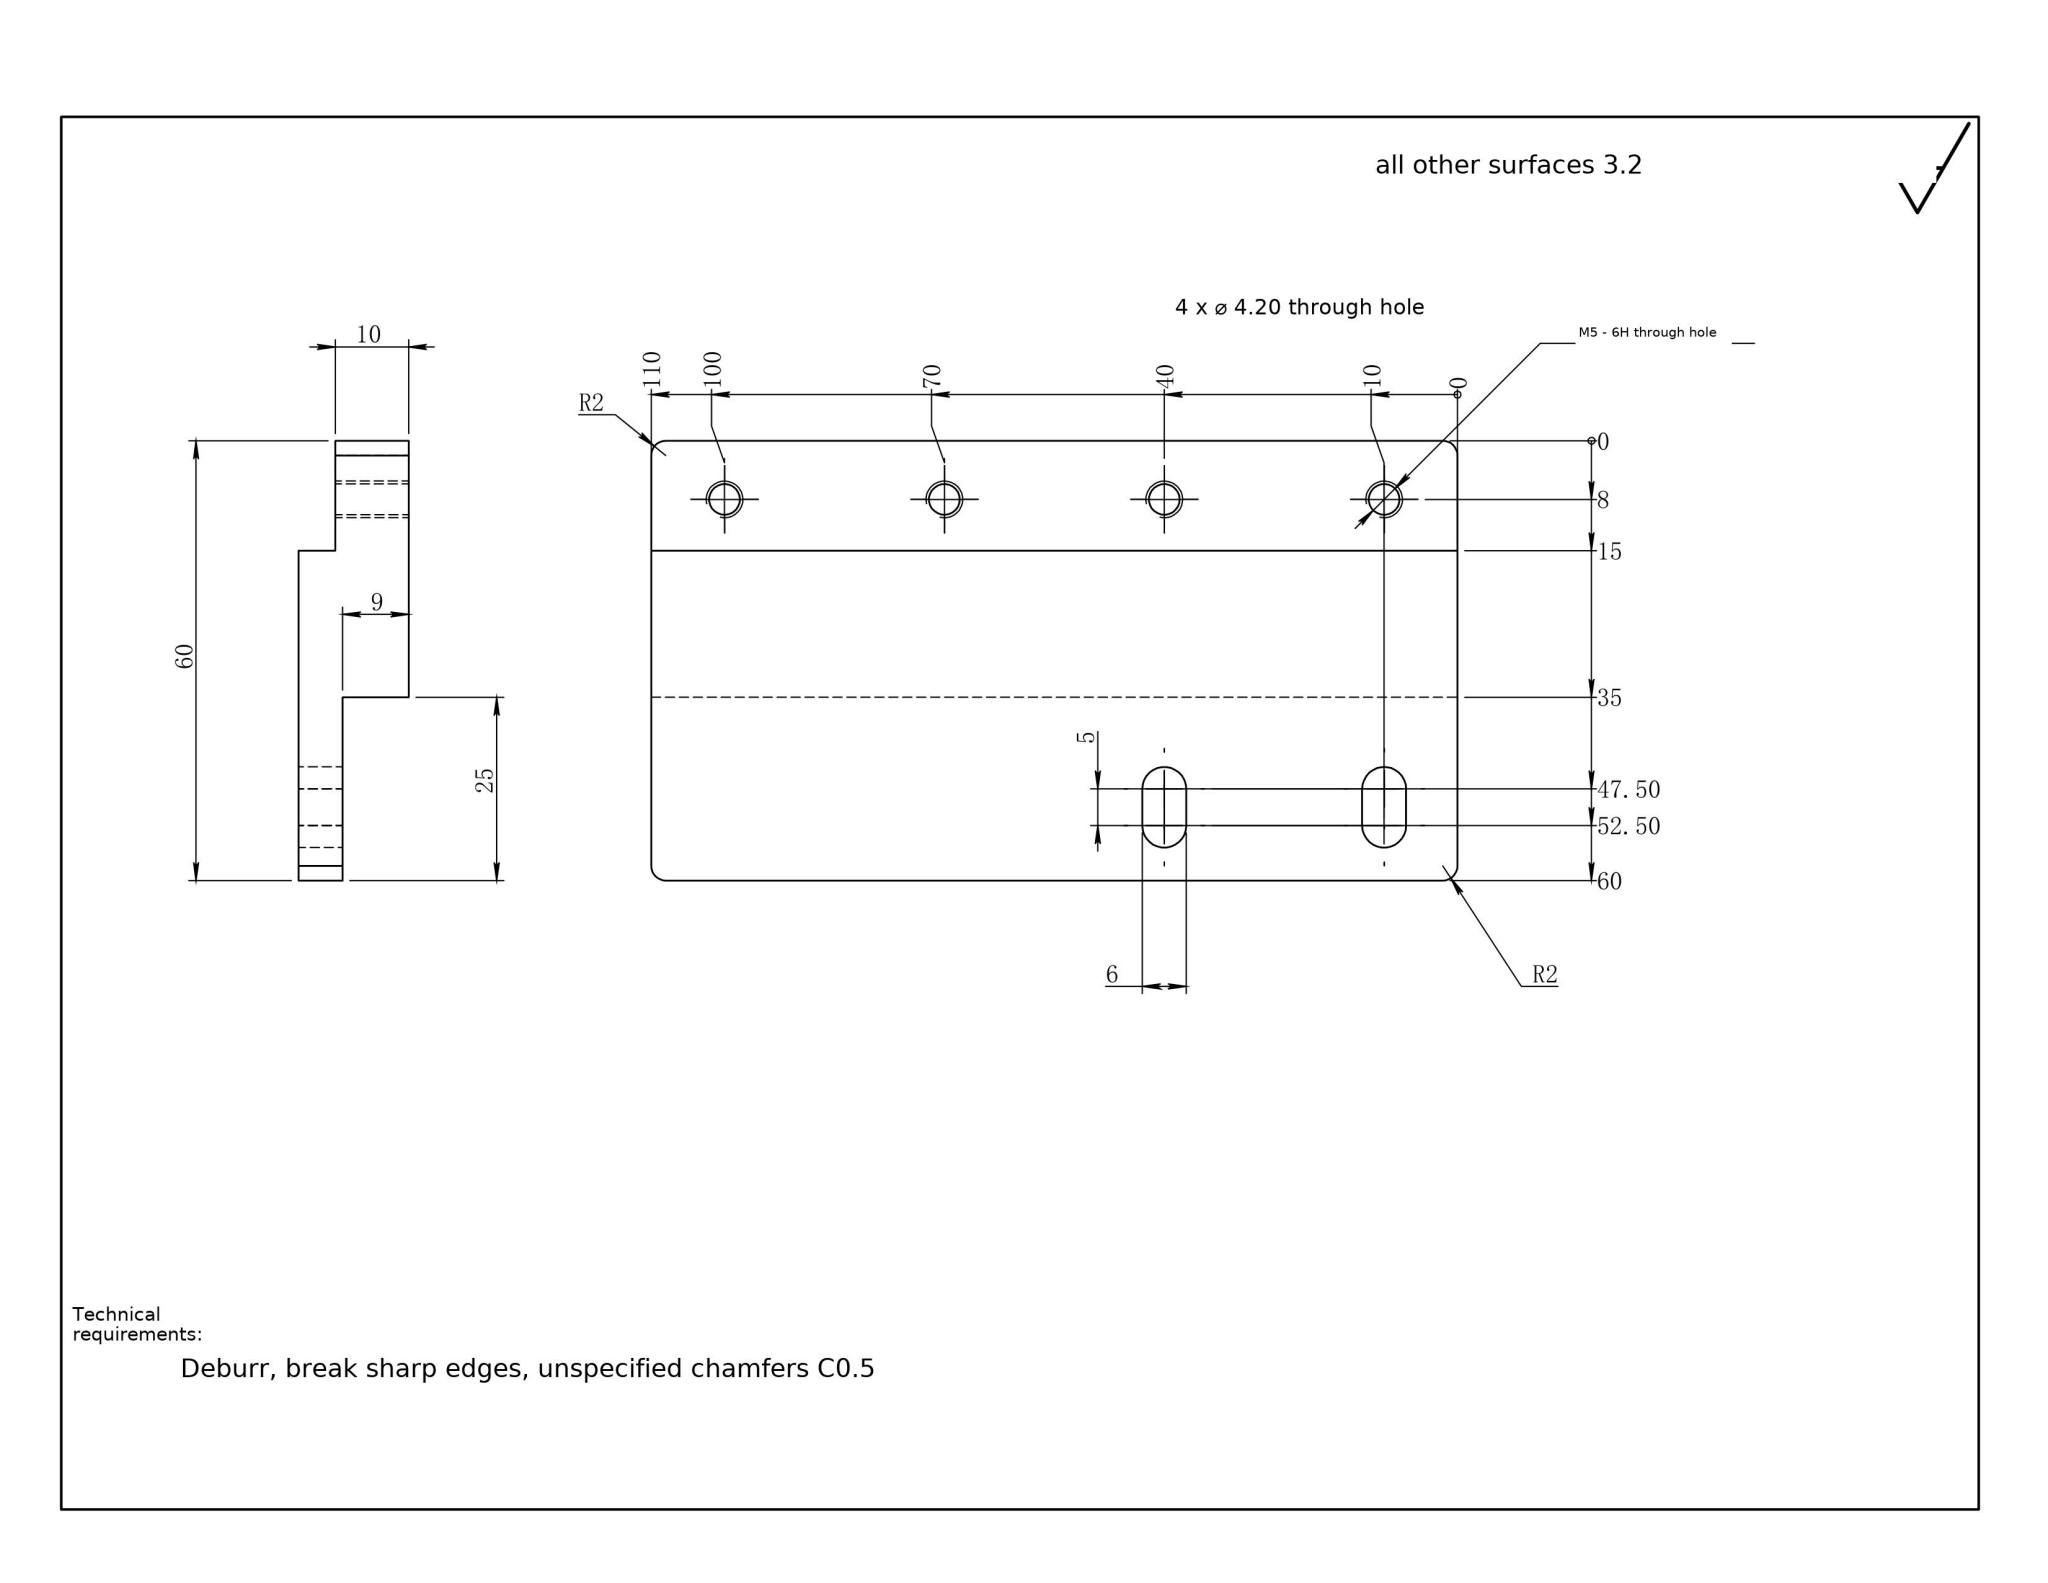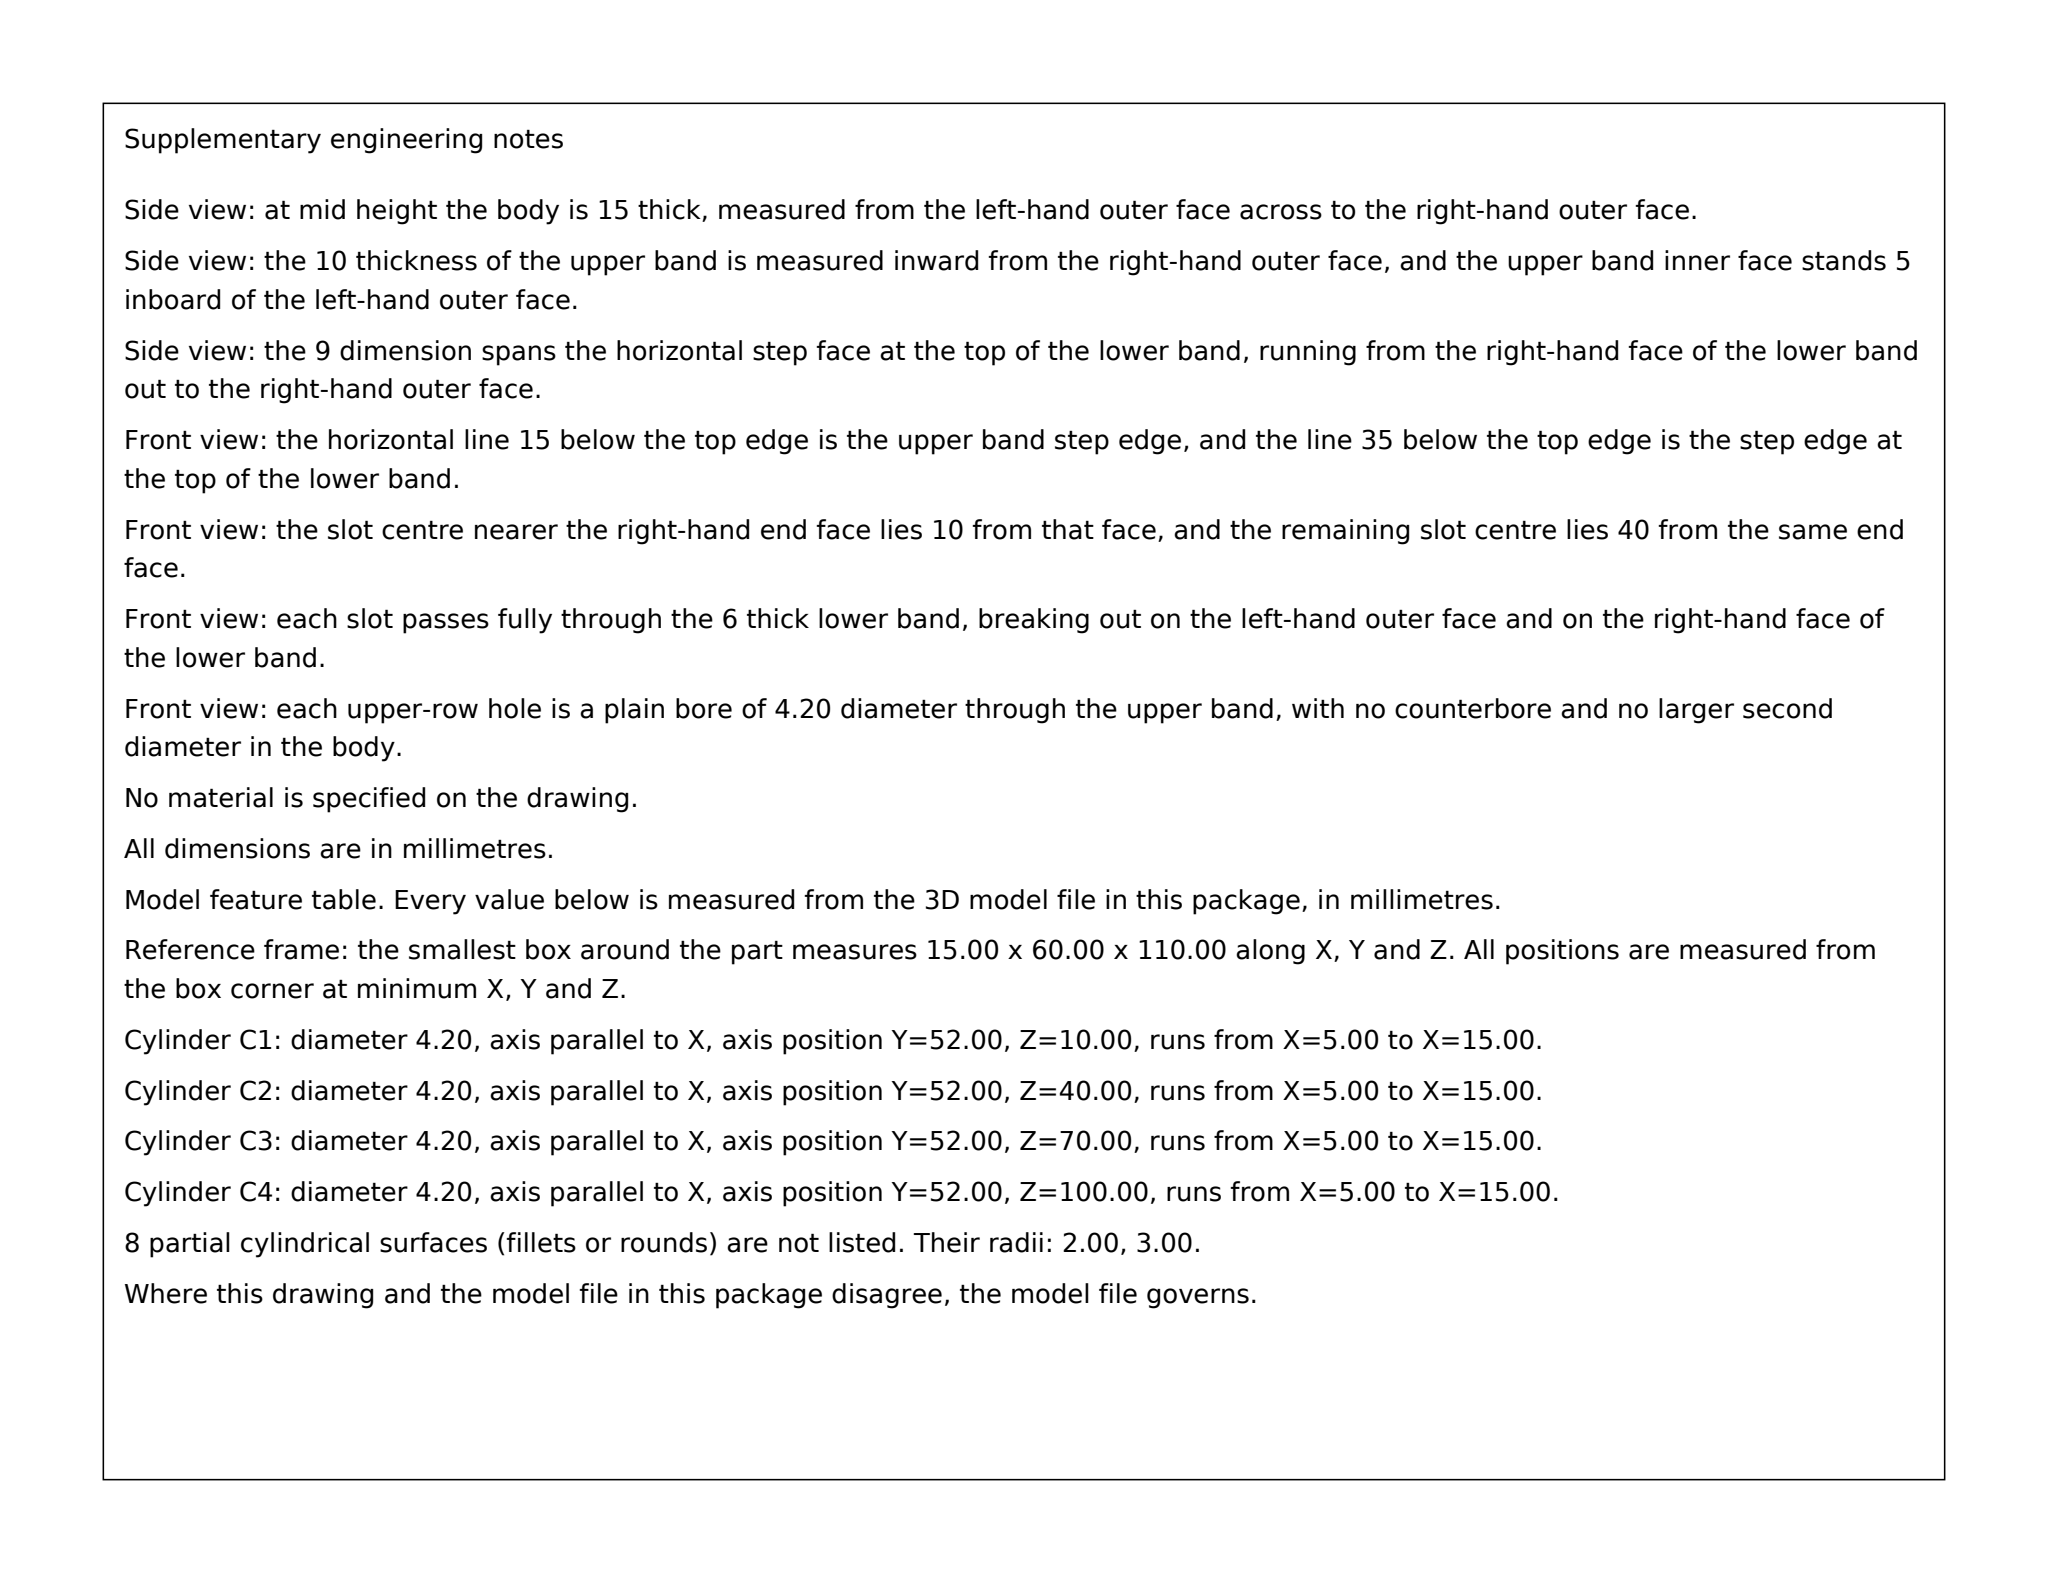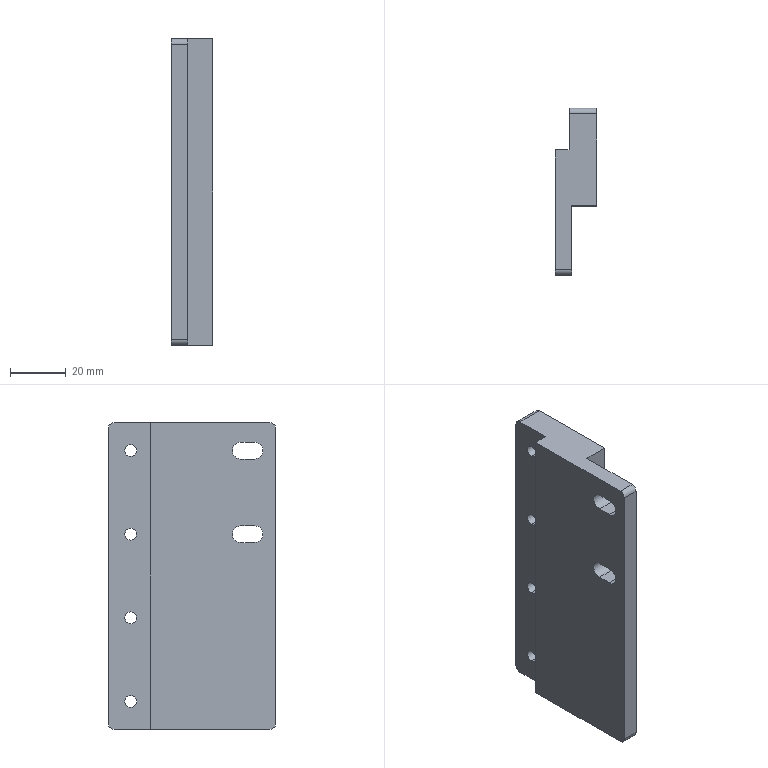Part | SolidWorks | mm | 1 solid | 30 faces | box 15 x 60 x 110 mm | volume 64719 mm3 | cylinder 16 | plane 14 | commonest cylinder face diameters 4.2 x8 4 x4 6 x4
Drawing notes:
OVERALL PART THICKNESS 15, MEASURED FROM BACK FACE (DATUM X0) TO FRONT FACE | from the solid: bbox_xyz x = 15.0; axis_planes x=0.0 and x=15.0
LOWER LIP (BOTTOM 25 HIGH FROM BOTTOM EDGE Y0) THICKNESS 6, FROM BACK FACE (DATUM X0) TO X6 | from the solid: axis_planes x=0.0, x=6.0, y=0.0, y=25.0; 6.0 dia slots length 6.0 at y=7.5/12.5
UPPER FLANGE (TOP PORTION CONTAINING THE 4X Ø4.20 HOLES) THICKNESS 10, FROM X5 TO FRONT FACE X15 | from the solid: axis_planes x=5.0 and x=15.0; 4.2 dia through holes length 10.0 at y=52.0
2X 6 WIDE OBROUND SLOT IN LOWER LIP: SLOT CENTRELINES AT Z70 AND Z100 FROM DATUM Z0 (RIGHT EDGE), COAXIAL IN Z WITH THE Ø4.20 HOLES AT 70 AND 100; SLOT THROUGH 6 DEEP FROM BACK FACE X0 TO X6. | from the solid: cylinders [6.0,"x",[null,7.5,70.0],6.0] and [6.0,"x",[null,12.5,70.0],6.0]; [6.0,"x",[null,7.5,100.0],6.0] and [6.0,"x",[null,12.5,100.0],6.0]; axis_plane x=6.0
build123d program:
from build123d import *

# Parameters (mm, degrees)
SKETCH1_W                = 110
SKETCH1_H                = 60
BOSS_EXTRUDE1_DEPTH      = 15
SKETCH2_W                = 9
SKETCH2_H                = 25
CUT_EXTRUDE1_DEPTH       = 116
M5_TAPPED_HOLE1_D        = 4.2
F_6_0_6_DIAMETER_HOLE1_D = 6
FILLET1_R                = 2
CUT_EXTRUDE2_DEPTH       = 65.42
SKETCH10_W               = 110
SKETCH10_H               = 15
CUT_EXTRUDE3_DEPTH       = 5


with BuildPart() as part:
    # Sketch1 → Boss-Extrude1 (new body)
    with BuildSketch(Plane(origin=(0, 0, 0), x_dir=(0, 0, -1), z_dir=(1, 0, 0))):
        Rectangle(SKETCH1_W, SKETCH1_H)
    extrude(amount=BOSS_EXTRUDE1_DEPTH)

    # Sketch2 → Cut-Extrude1 (cut, through all)
    with BuildSketch(Plane.XY.offset(55)):
        with Locations((10.5, -17.5)):
            Rectangle(SKETCH2_W, SKETCH2_H)
    extrude(amount=-CUT_EXTRUDE1_DEPTH, mode=Mode.SUBTRACT)

    # M5 Tapped Hole1 (through all)
    with Locations(Plane.ZY):
        with Locations((45, 22), (15, 22), (-15, 22), (-45, 22)):
            Hole(M5_TAPPED_HOLE1_D / 2)

    # 6.0 _6_ Diameter Hole1 (through all)
    with Locations(Plane.ZY):
        with Locations((45, -20), (15, -20)):
            Hole(F_6_0_6_DIAMETER_HOLE1_D / 2)

    # Fillet1
    fillet1_edges = [part.edges().sort_by_distance(p)[0] for p in [
        (3, -30, -55),
        (3, -30, 55),
        (7.5, 30, 55),
        (7.5, 30, -55),
    ]]
    fillet(fillet1_edges, radius=FILLET1_R)

    # Sketch9 → Cut-Extrude2 (cut, through all)
    with BuildSketch(Plane.ZY):
        with BuildLine():
            Line((12, -22.5), (12, -17.5))
            ThreePointArc((12, -17.5), (15, -14.5), (18, -17.5))
            Line((18, -17.5), (18, -22.5))
            ThreePointArc((18, -22.5), (15, -25.5), (12, -22.5))
        make_face()
        with BuildLine():
            Line((42, -22.5), (42, -17.5))
            ThreePointArc((42, -17.5), (45, -14.5), (48, -17.5))
            Line((48, -17.5), (48, -22.5))
            ThreePointArc((48, -22.5), (45, -25.5), (42, -22.5))
        make_face()
    extrude(amount=-CUT_EXTRUDE2_DEPTH, mode=Mode.SUBTRACT)

    # Sketch10 → Cut-Extrude3 (cut)
    with BuildSketch(Plane.ZY):
        with Locations((0, 22.5)):
            Rectangle(SKETCH10_W, SKETCH10_H)
    extrude(amount=-CUT_EXTRUDE3_DEPTH, mode=Mode.SUBTRACT)


solid = part.part